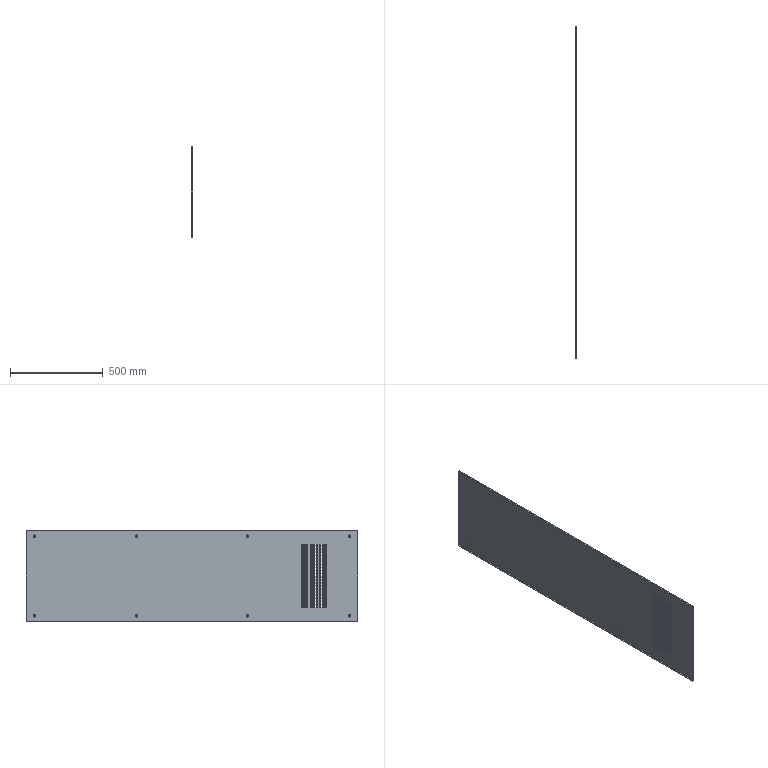Component | SolidWorks | KSHE-016.019-1 | 1 solid | 686 faces | volume 1077457 mm3 | plane 566 | torus 64 | cylinder 56 | commonest cylinder face diameters 9.6 x16 12 x16 6 x16 2.6 x4 0.2 x4